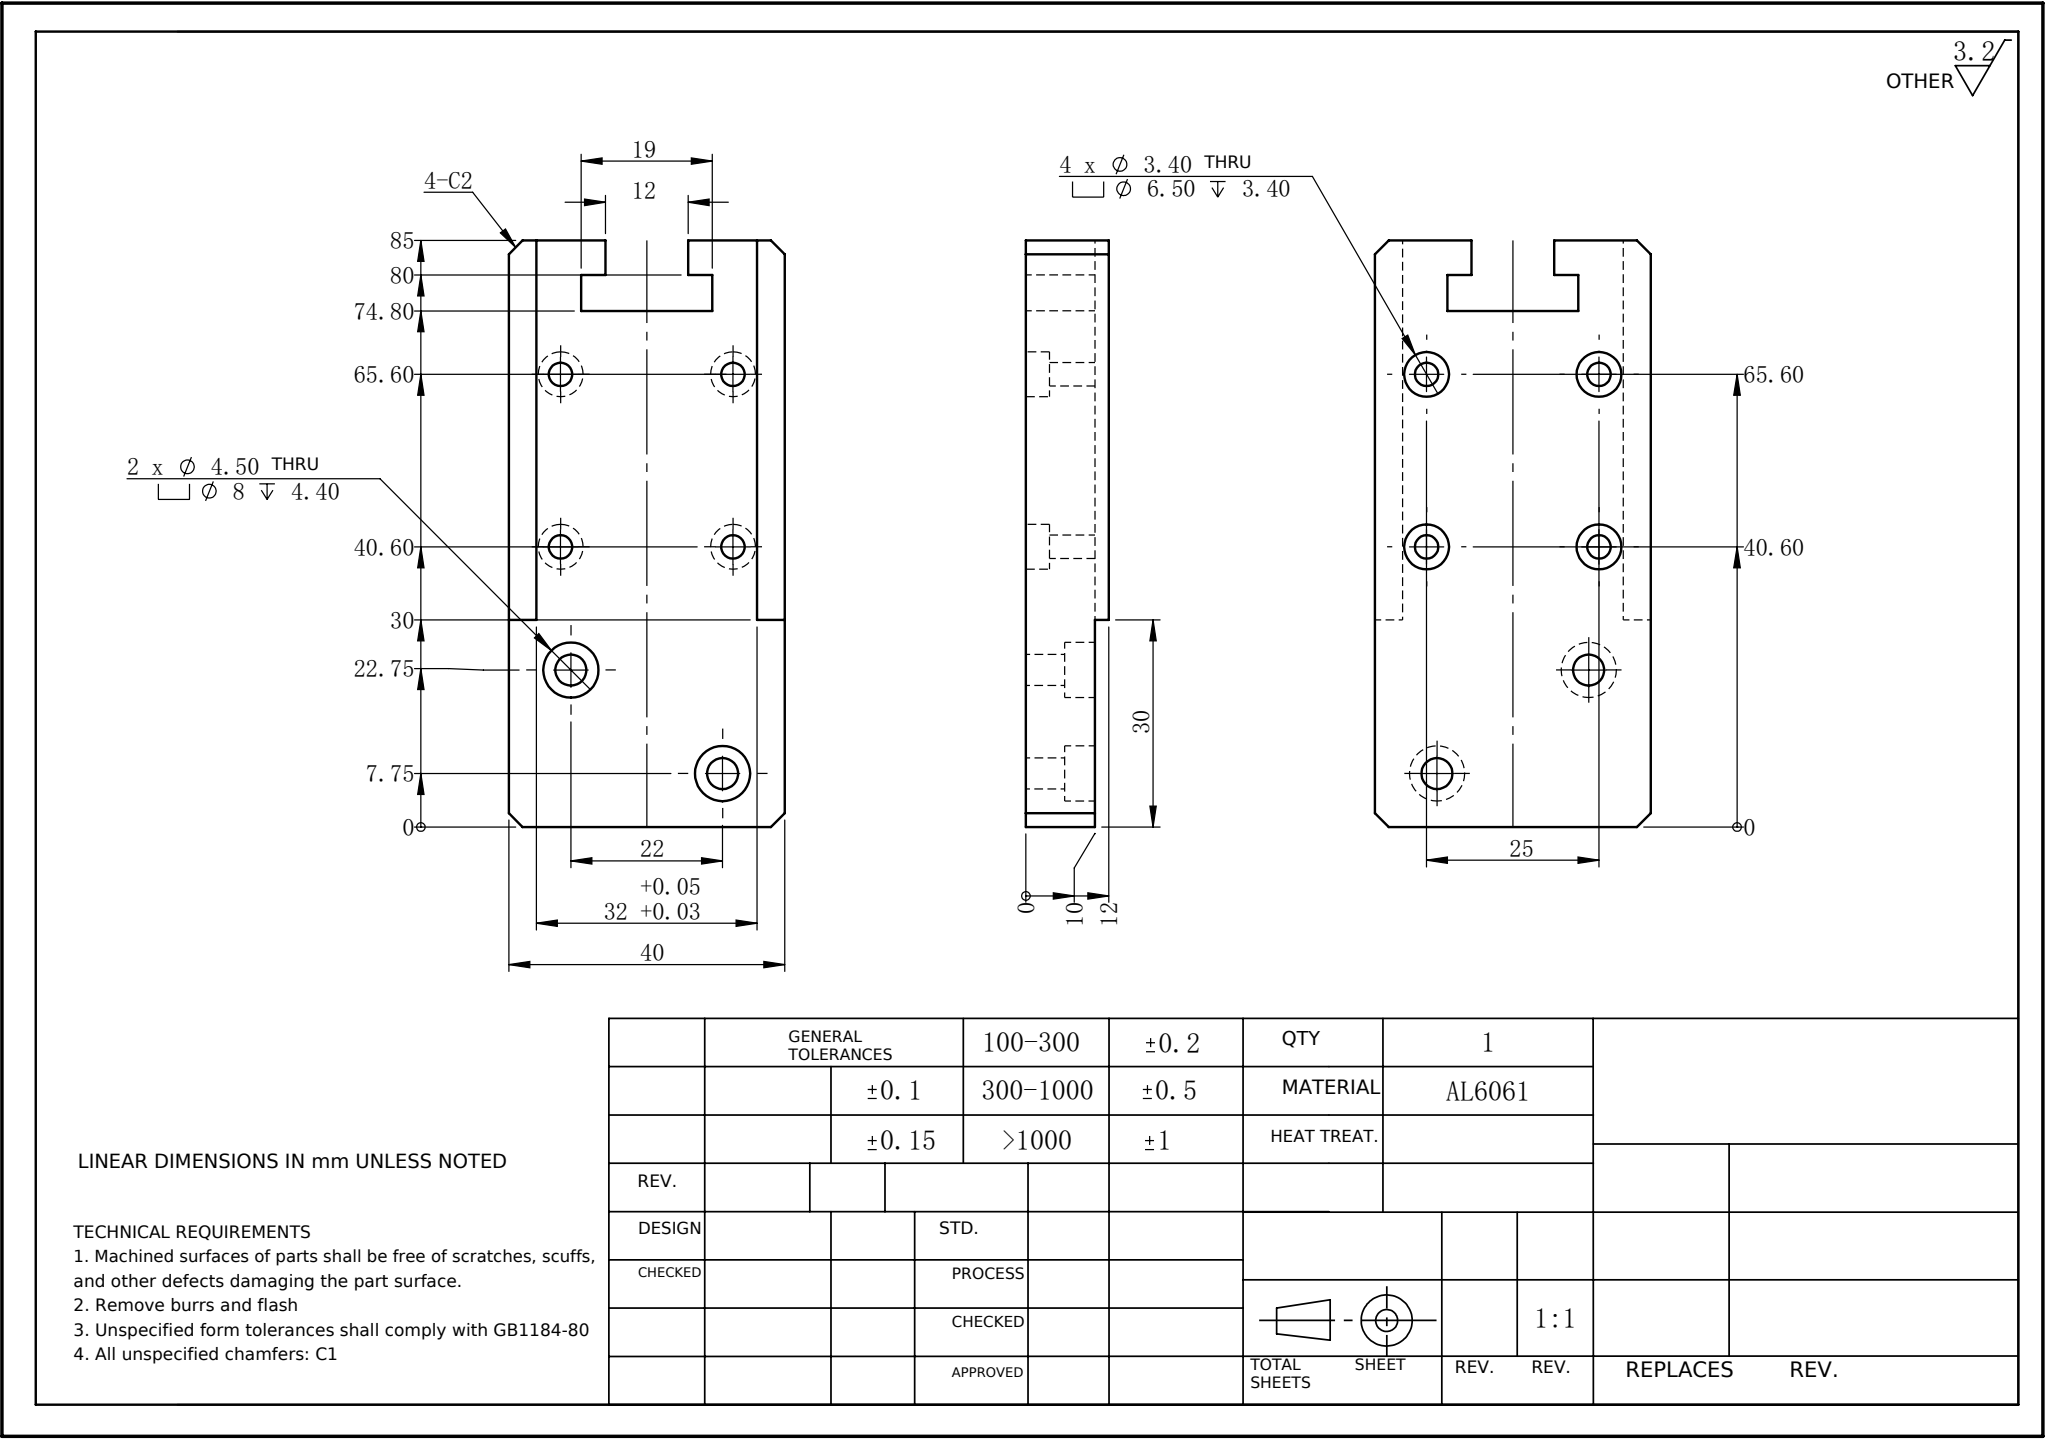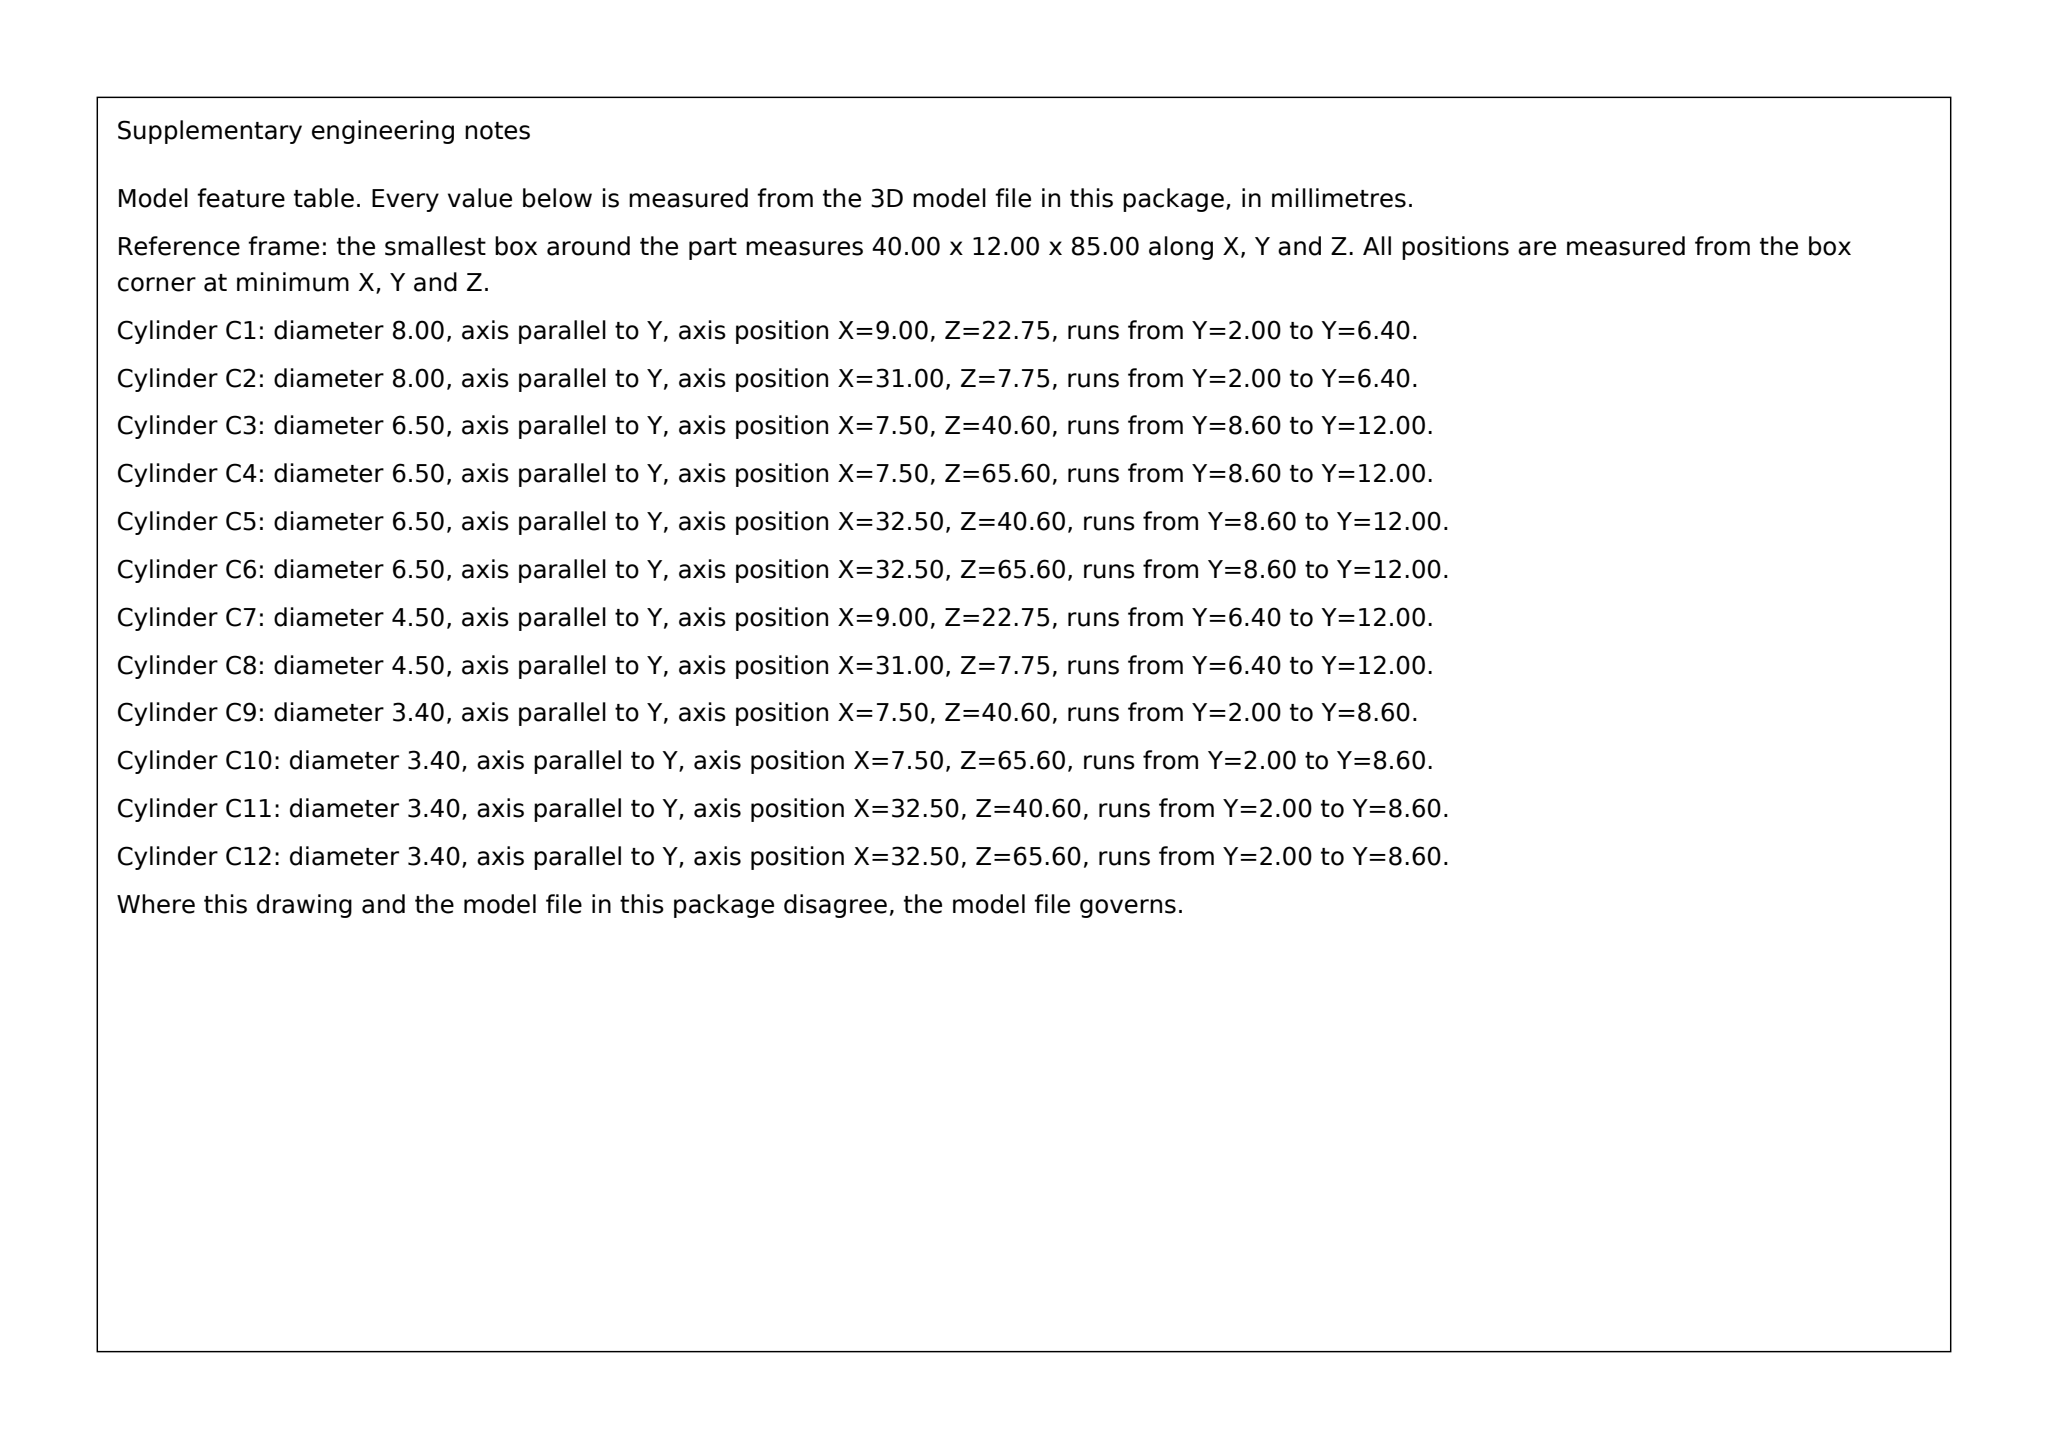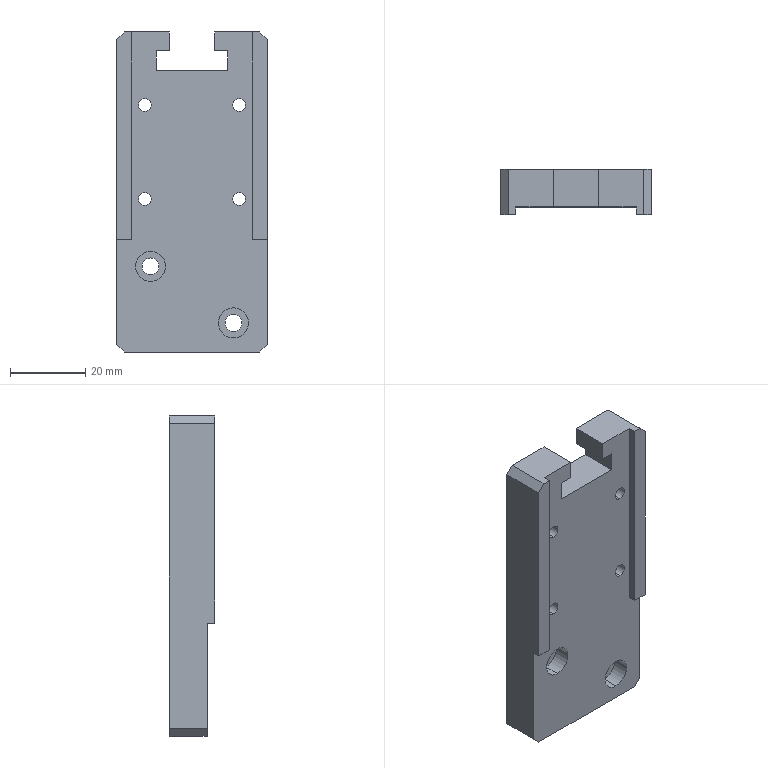Part | SolidWorks | mm | material AL6061 | 1 solid | 54 faces | box 40 x 12 x 85 mm | volume 31893 mm3 | plane 30 | cylinder 24 | commonest cylinder face diameters 6.5 x8 3.4 x8 8 x4 4.5 x4
build123d program:
from build123d import *

# Parameters (mm, degrees)
SKETCH1_W                                       = 40
SKETCH1_H                                       = 85
BOSS_EXTRUDE1_DEPTH                             = 5
M3_HEX_SOCKET_HEAD_CAP_SCREW_CBORE1_D           = 3.4
M3_HEX_SOCKET_HEAD_CAP_SCREW_CBORE1_CBORE_D     = 6.5
M3_HEX_SOCKET_HEAD_CAP_SCREW_CBORE1_CBORE_DEPTH = 3.4
M4_HEX_SOCKET_HEAD_CAP_SCREW_CBORE1_D           = 4.5
M4_HEX_SOCKET_HEAD_CAP_SCREW_CBORE1_CBORE_D     = 8
M4_HEX_SOCKET_HEAD_CAP_SCREW_CBORE1_CBORE_DEPTH = 4.4
SKETCH6_W                                       = 4
SKETCH6_H                                       = 55
BOSS_EXTRUDE2_DEPTH                             = 2
CHAMFER1_SIZE                                   = 2
SKETCH7_W                                       = 12
SKETCH7_H                                       = 10
CUT_EXTRUDE1_DEPTH                              = 14
SKETCH8_W                                       = 19
SKETCH8_H                                       = 5.2
CUT_EXTRUDE2_DEPTH                              = 14


with BuildPart() as part:
    # Sketch1 → Boss-Extrude1 (new, symmetric)
    with BuildSketch(Plane(origin=(0, 0, 0), x_dir=(1, 0, 0), z_dir=(0, 1, 0))):
        Rectangle(SKETCH1_W, SKETCH1_H)
    extrude(amount=BOSS_EXTRUDE1_DEPTH, both=True)

    # M3 Hex Socket Head Cap Screw CBORE1 (through all)
    with Locations(Plane(origin=(0, 5, 0), x_dir=(1, 0, 0), z_dir=(0, 1, 0))):
        with Locations((-12.5, -23.1), (-12.5, 1.9), (12.5, 1.9), (12.5, -23.1)):
            CounterBoreHole(M3_HEX_SOCKET_HEAD_CAP_SCREW_CBORE1_D / 2, M3_HEX_SOCKET_HEAD_CAP_SCREW_CBORE1_CBORE_D / 2, M3_HEX_SOCKET_HEAD_CAP_SCREW_CBORE1_CBORE_DEPTH)

    # M4 Hex Socket Head Cap Screw CBORE1 (through all)
    with Locations(Plane(origin=(0, -5, 0), x_dir=(-1, 0, 0), z_dir=(0, -1, 0))):
        with Locations((-11, 34.75), (11, 19.75)):
            CounterBoreHole(M4_HEX_SOCKET_HEAD_CAP_SCREW_CBORE1_D / 2, M4_HEX_SOCKET_HEAD_CAP_SCREW_CBORE1_CBORE_D / 2, M4_HEX_SOCKET_HEAD_CAP_SCREW_CBORE1_CBORE_DEPTH)

    # Sketch6 → Boss-Extrude2 (add)
    with BuildSketch(Plane.XZ.offset(5)):
        with Locations((18, 15)):
            Rectangle(SKETCH6_W, SKETCH6_H)
        with Locations((-18, 15)):
            Rectangle(SKETCH6_W, SKETCH6_H)
    extrude(amount=BOSS_EXTRUDE2_DEPTH)

    # Chamfer1
    chamfer1_edges = [part.edges().sort_by_distance(p)[0] for p in [
        (20, -1, 42.5),
        (-20, -1, 42.5),
        (-20, 0, -42.5),
        (20, 0, -42.5),
    ]]
    chamfer(chamfer1_edges, length=CHAMFER1_SIZE)

    # Sketch7 → Cut-Extrude1 (cut)
    with BuildSketch(Plane(origin=(0, 5, 0), x_dir=(1, 0, 0), z_dir=(0, 1, 0))):
        with Locations((0, -42.5)):
            Rectangle(SKETCH7_W, SKETCH7_H)
    extrude(amount=-CUT_EXTRUDE1_DEPTH, mode=Mode.SUBTRACT)

    # Sketch8 → Cut-Extrude2 (cut)
    with BuildSketch(Plane(origin=(0, 5, 0), x_dir=(1, 0, 0), z_dir=(0, 1, 0))):
        with Locations((0, -34.9)):
            Rectangle(SKETCH8_W, SKETCH8_H)
    extrude(amount=-CUT_EXTRUDE2_DEPTH, mode=Mode.SUBTRACT)


solid = part.part